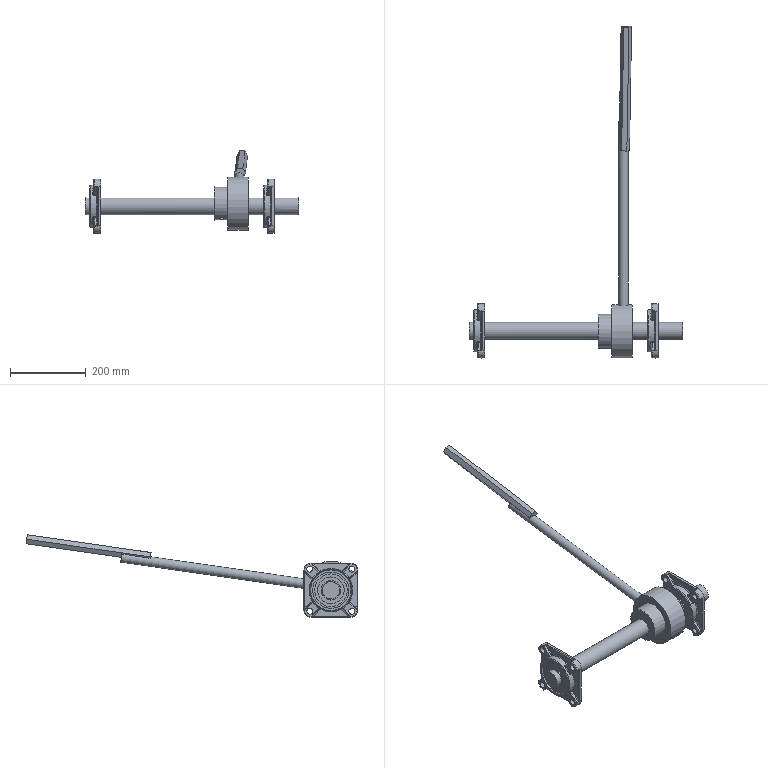Assembly | NX | mm | 9 component files | 9 solids | 536 faces | box 565 x 876.73 x 218.01 mm | volume 2548543 mm3 | cylinder 185 | plane 168 | spline 96 | torus 54 | sphere 32 | cone 1 | commonest cylinder face diameters 4 x80 20 x16 16 x8 40 x8 143 x8 51 x4 45 x4 115 x3
Bill of materials:
unnamed part 1 | 1 |  | Thin flat split ring of roughly constant radial width. At the split, two short lugs stick out past the outer edge, and each lug has a small round hole. The gap between the lugs is narrow.
unnamed part 2 | 1 |  | Flat annular ring (washer-like) with a rectangular cross-section and rounded or slightly chamfered edges. It is fairly thick relative to its radial width.
unnamed part 3 | 1 |  | Long straight prismatic bar with a faceted cross-section that looks partly hexagonal. A concave, arc-shaped channel runs along one side for the full length. A small step or offset is visible partway along one edge.
unnamed part 4 | 1 |  | Thin flat open ring with a wide gap. The radial width tapers, widest opposite the gap and narrower near the ends. Each end has a lug that turns inward with a small round hole.
unnamed part 5 | 1 |  | Short, thick-walled cylindrical ring (eye) with a long, thin, straight round rod attached radially to its outside. The rod is much narrower than the ring is wide.
unnamed part 6 | 1 |  | Plain, solid, straight cylindrical rod with flat ends. A small notch or flat sits on one edge of the end face.
unnamed part 7 | 1 |  | Square plate flange with rounded corners. It has four corner through-holes, a central circular through-bore, and a cross-shaped raised or recessed pad with filleted contours on the front face. A stepped circular boss or spigot projects from the back.
unnamed part 8 | 1 |  | Square plate flange with rounded corners. It has four corner through-holes, a central circular through-bore, and a cross-shaped raised or recessed pad with filleted contours on the front face. A stepped circular boss or spigot projects from the back.
unnamed part 9 | 1 |  | Stepped cylindrical sleeve or bushing with a larger-diameter section, a shoulder, and a smaller-diameter section. A through-bore runs the length, and a narrow groove sits near the end of the smaller section. A small radial hole is visible on the larger section.
Mates:
1. touch align | hex_steel 1 face | drive_rod 1 face